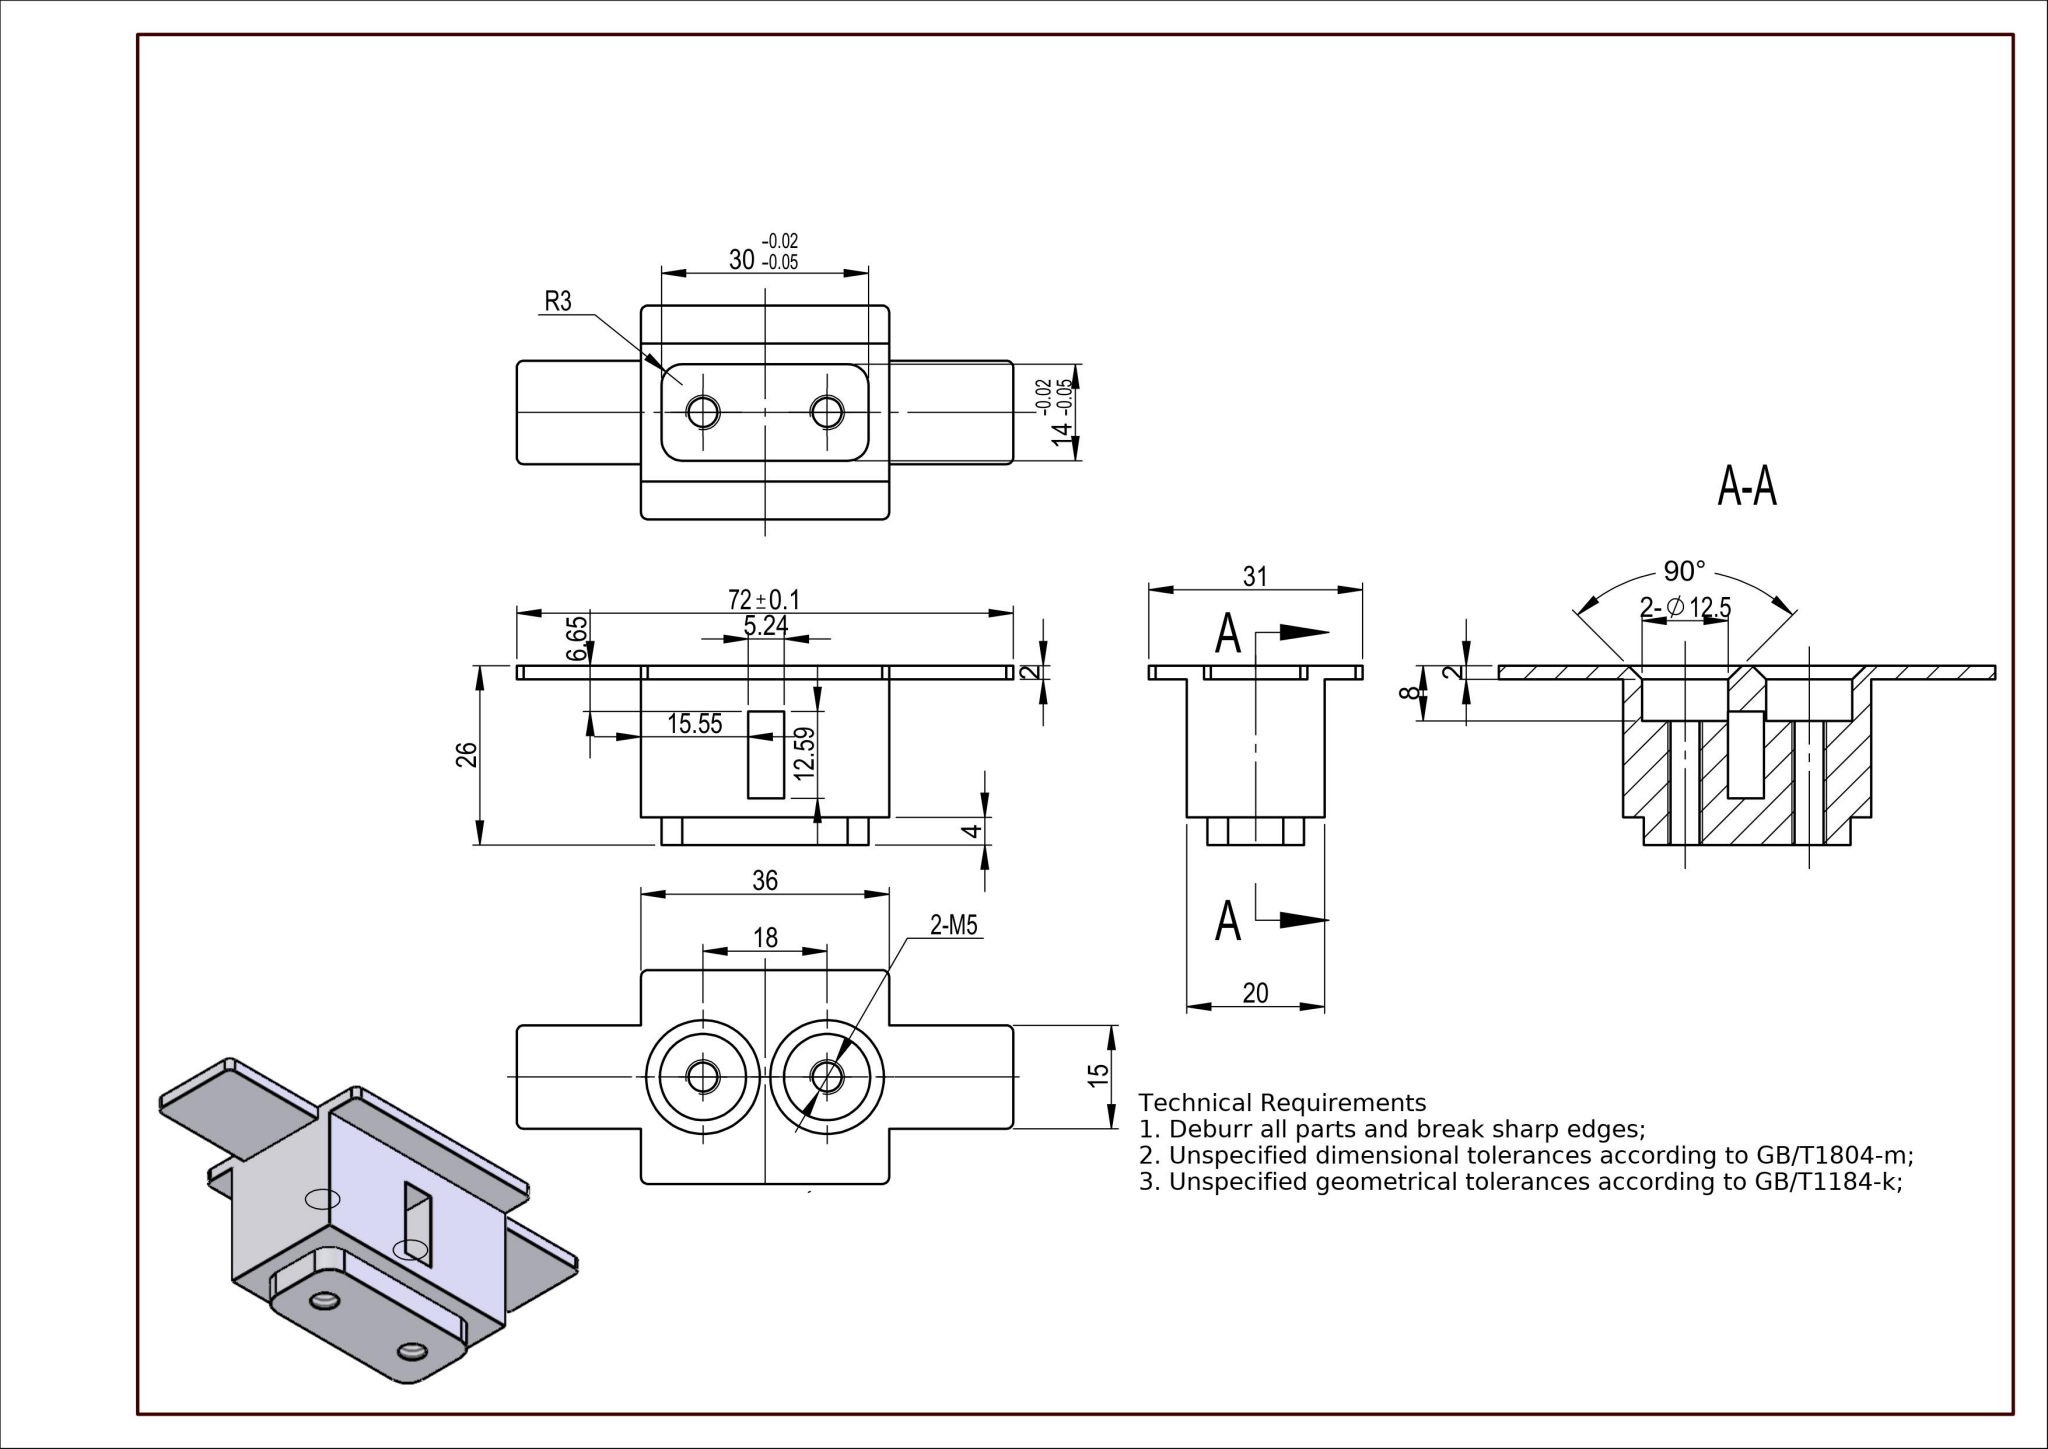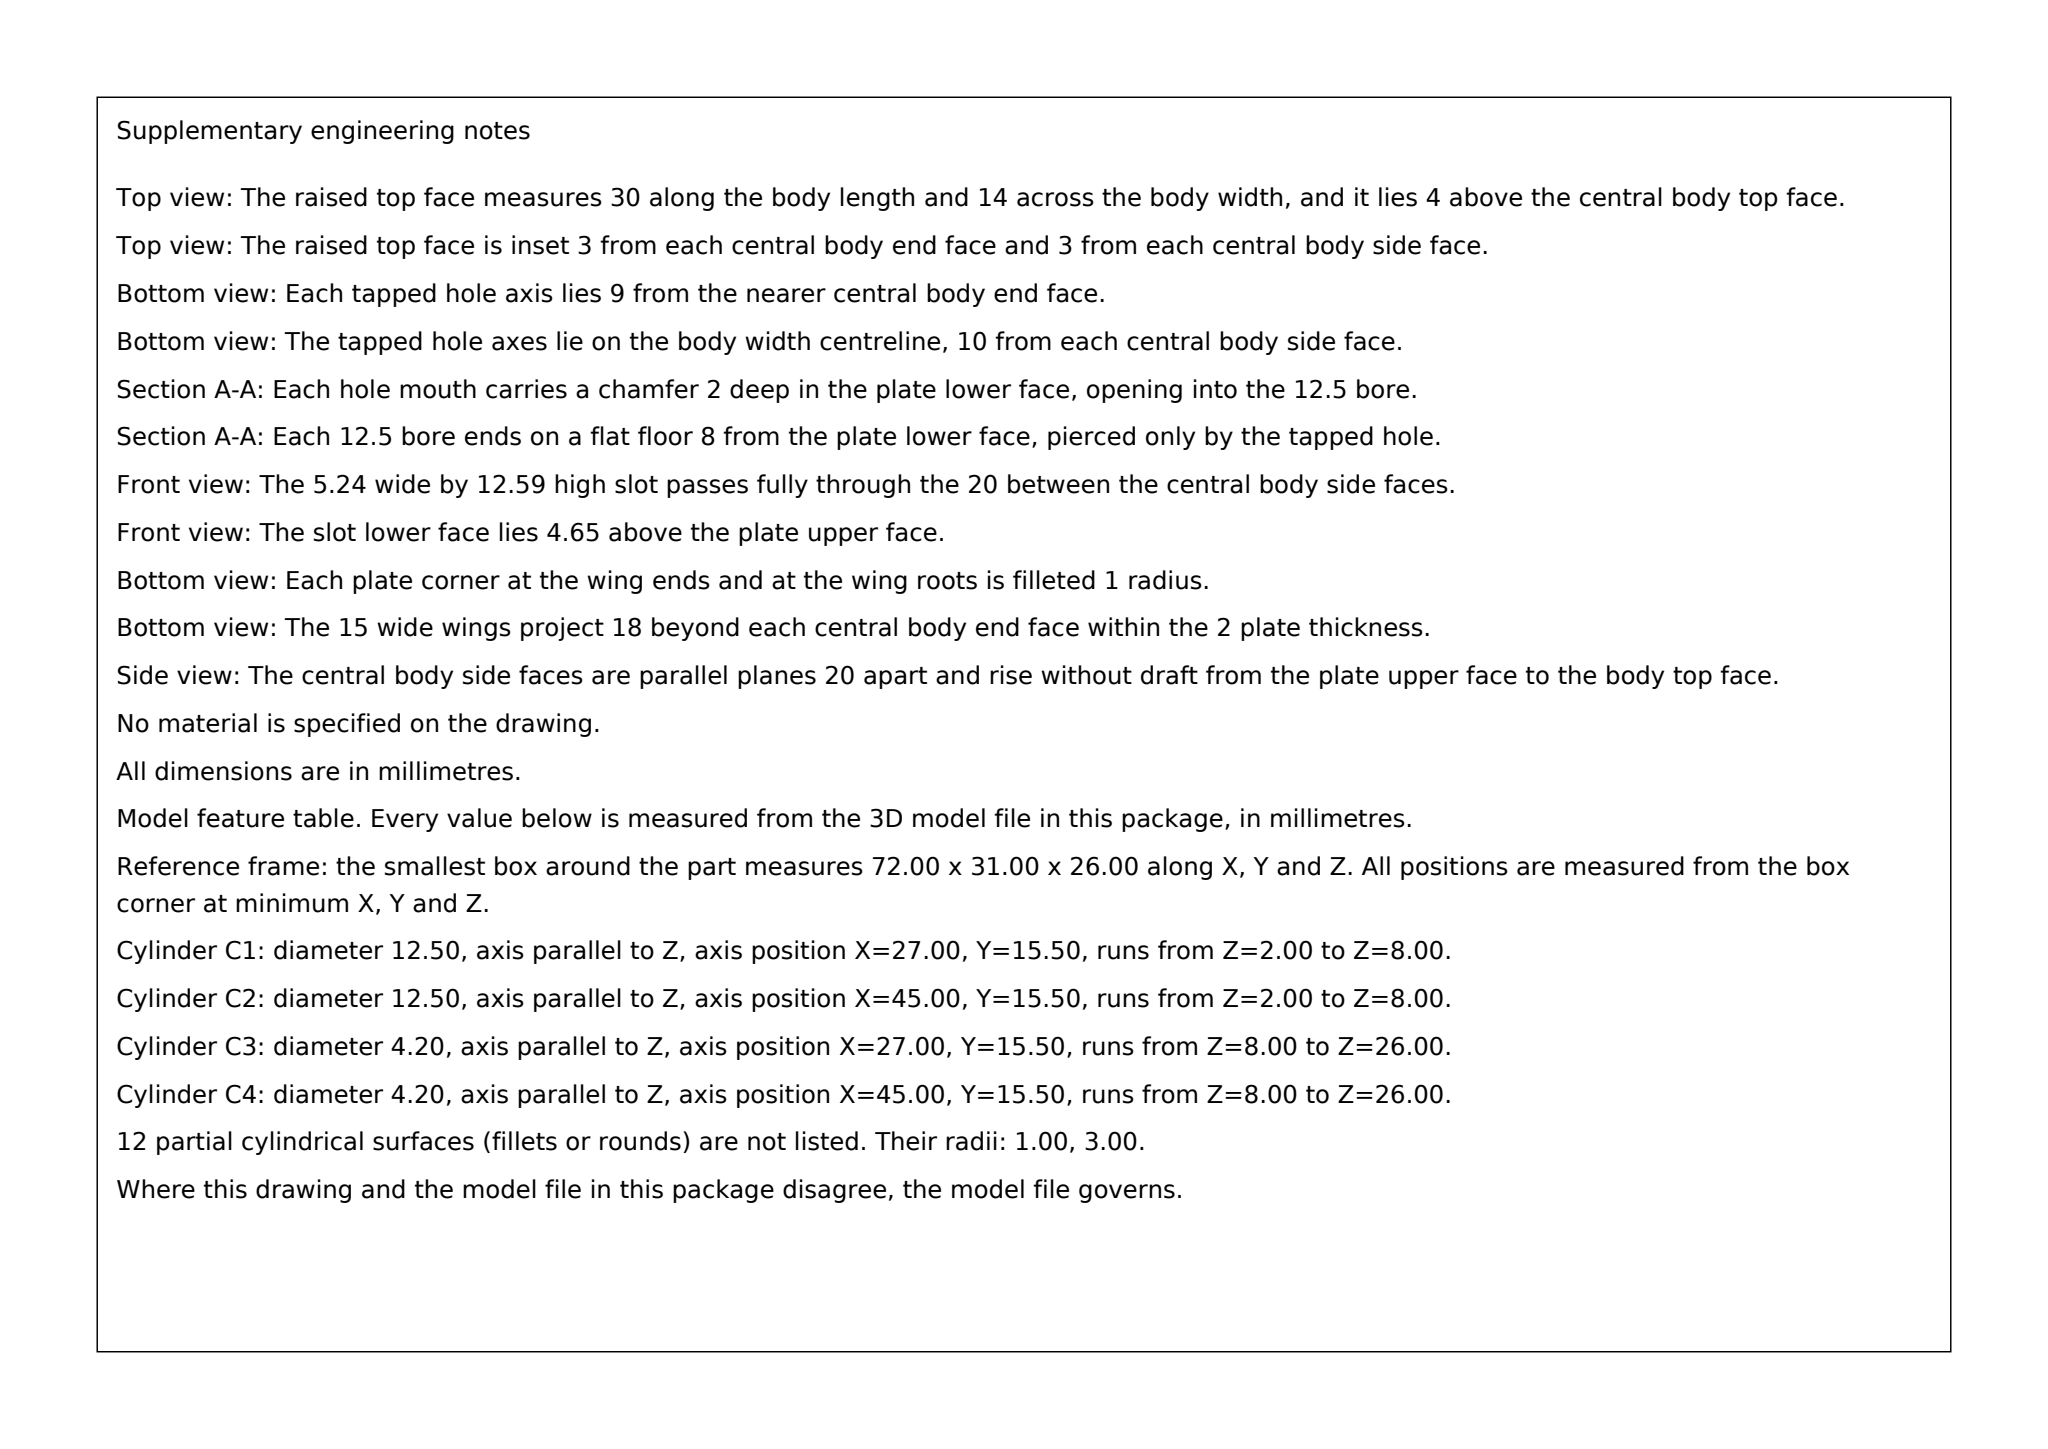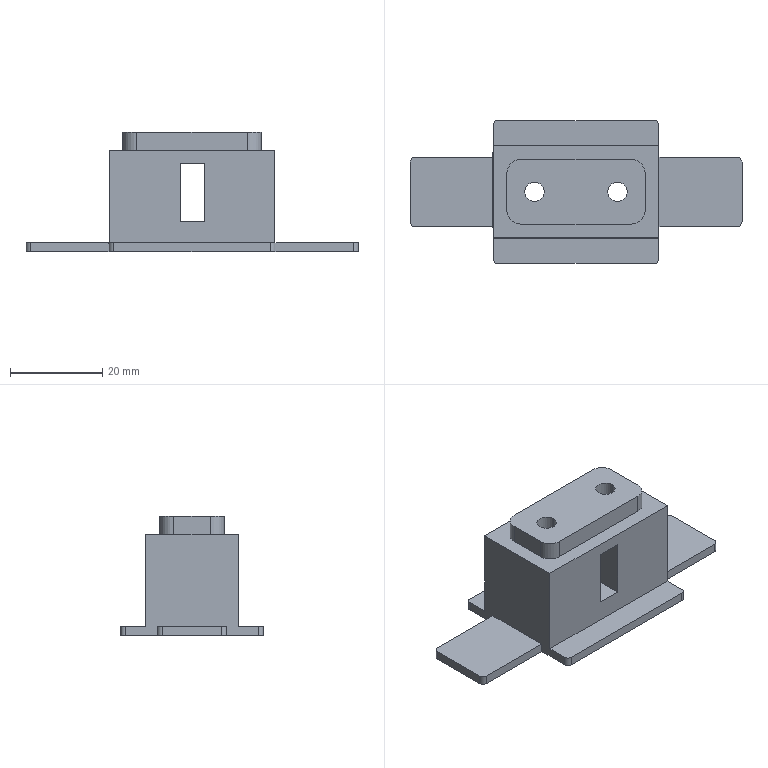Part | SolidWorks | mm | 1 solid | 53 faces | box 72 x 31 x 26 mm | volume 15402 mm3 | plane 29 | cylinder 20 | cone 4 | commonest cylinder face diameters 2 x8 4.2 x4 12.5 x4 6 x4
Drawing notes:
4X Ø6 BOSS DP 4 ON BOTTOM FACE (SEE A-A) | from the solid: cylinders dia 6.0, axis z, length 4.0, count 4 at z=0..4
Ø6 BOSSES SPACED 24 X 8, SYM ABOUT BOTH CENTERLINES | from the solid: boss centers x=24/48 (±12 of 36), y=11.5/19.5 (±4 of 15.5)
2-M5: Ø4.2 DRILL DP 18, NOT THRU; SPACED 18 | from the solid: cylinders dia 4.2, axis z, length 18.0 at x=27/45, y=15.5; part height 26
8X Ø2 BOSS, 2 DEEP (R1 CORNER PADS) ON TOP FLANGE FACE (Z=0 TO 2); CENTERS AT X/Y FROM BBOX MIN CORNER: (1,9), (1,22), (19,1), (19,30), (53,1), (53,30), (71,9), (71,22) | from the solid: cylinders dia 2.0, axis z, length 2.0, count 8 at listed positions
8X R1 (Ø2) corner fillets on 2 mm flange plate; fillet centers at X/Y = (1,9), (1,22), (19,1), (19,30), (53,1), (53,30), (71,9), (71,22) from bbox min corner, through 2 mm plate thickness | from the solid: cylinders dia 2.0, axis z, length 2.0, 8 instances at [1,9],[1,22],[19,1],[19,30],[53,1],[53,30],[71,9],[71,22]
build123d program:
from build123d import *

# Parameters (mm, degrees)
SKETCH1_W           = 36
SKETCH1_H           = 31
BOSS_EXTRUDE1_DEPTH = 1
SKETCH2_W           = 36
SKETCH2_H           = 20
BOSS_EXTRUDE2_DEPTH = 20
SKETCH3_W           = 30
SKETCH3_H           = 14
BOSS_EXTRUDE3_DEPTH = 4
FILLET1_R           = 3
SKETCH4_R           = 6.25
CUT_EXTRUDE1_DEPTH  = 8
CHAMFER1_SIZE       = 2
M5_TAPPED_HOLE1_D   = 4.2
SKETCH8_W           = 2
SKETCH8_H           = 15
BOSS_EXTRUDE4_DEPTH = 18
FILLET2_R           = 1
SKETCH11_W          = 5.241
SKETCH11_H          = 12.591
CUT_EXTRUDE2_DEPTH  = 58


with BuildPart() as part:
    # Sketch1 → Boss-Extrude1 (new, symmetric)
    with BuildSketch(Plane.XY):
        Rectangle(SKETCH1_W, SKETCH1_H)
    extrude(amount=BOSS_EXTRUDE1_DEPTH, both=True)

    # Sketch2 → Boss-Extrude2 (add)
    with BuildSketch(Plane.XY.offset(1)):
        Rectangle(SKETCH2_W, SKETCH2_H)
    extrude(amount=BOSS_EXTRUDE2_DEPTH)

    # Sketch3 → Boss-Extrude3 (add)
    with BuildSketch(Plane.XY.offset(21)):
        Rectangle(SKETCH3_W, SKETCH3_H)
    extrude(amount=BOSS_EXTRUDE3_DEPTH)

    # Fillet1
    fillet1_edges = [part.edges().sort_by_distance(p)[0] for p in [
        (15, -7, 23),
        (15, 7, 23),
        (-15, 7, 23),
        (-15, -7, 23),
    ]]
    fillet(fillet1_edges, radius=FILLET1_R)

    # Sketch4 → Cut-Extrude1 (cut)
    with BuildSketch(Plane(origin=(0, 0, -1), x_dir=(-1, 0, 0), z_dir=(0, 0, -1))):
        with Locations((9, 0)):
            Circle(SKETCH4_R)
        with Locations((-9, 0)):
            Circle(SKETCH4_R)
    extrude(amount=-CUT_EXTRUDE1_DEPTH, mode=Mode.SUBTRACT)

    # Chamfer1
    chamfer1_edges = [part.edges().sort_by_distance(p)[0] for p in [
        (-2.75, 0, -1),
        (15.25, 0, -1),
    ]]
    chamfer(chamfer1_edges, length=CHAMFER1_SIZE)

    # M5 Tapped Hole1 (through all)
    with Locations(Plane(origin=(0, 0, 7), x_dir=(-1, 0, 0), z_dir=(0, 0, -1))):
        with Locations((9, 0), (-9, 0)):
            Hole(M5_TAPPED_HOLE1_D / 2)

    # Sketch8 → Boss-Extrude4 (add)
    with BuildSketch(Plane(origin=(18, 0, 0), x_dir=(0, 0, -1), z_dir=(1, 0, 0))):
        Rectangle(SKETCH8_W, SKETCH8_H)
    boss_extrude4 = extrude(amount=BOSS_EXTRUDE4_DEPTH)

    # Mirror1: Boss-Extrude4 across plane
    add(boss_extrude4.mirror(Plane(origin=(0, 0, 0), x_dir=(0, 0, 1), z_dir=(1, 0, 0))))

    # Fillet2
    fillet2_edges = [part.edges().sort_by_distance(p)[0] for p in [
        (-18, -15.5, 0),
        (-18, 15.5, 0),
        (18, 15.5, 0),
        (18, -15.5, 0),
        (36, -7.5, 0),
        (36, 7.5, 0),
        (-36, 7.5, 0),
        (-36, -7.5, 0),
    ]]
    fillet(fillet2_edges, radius=FILLET2_R)

    # Sketch11 → Cut-Extrude2 (cut)
    with BuildSketch(Plane.XZ.offset(10)):
        with Locations((0.1709, 11.943)):
            Rectangle(SKETCH11_W, SKETCH11_H)
    extrude(amount=-CUT_EXTRUDE2_DEPTH, mode=Mode.SUBTRACT)


solid = part.part